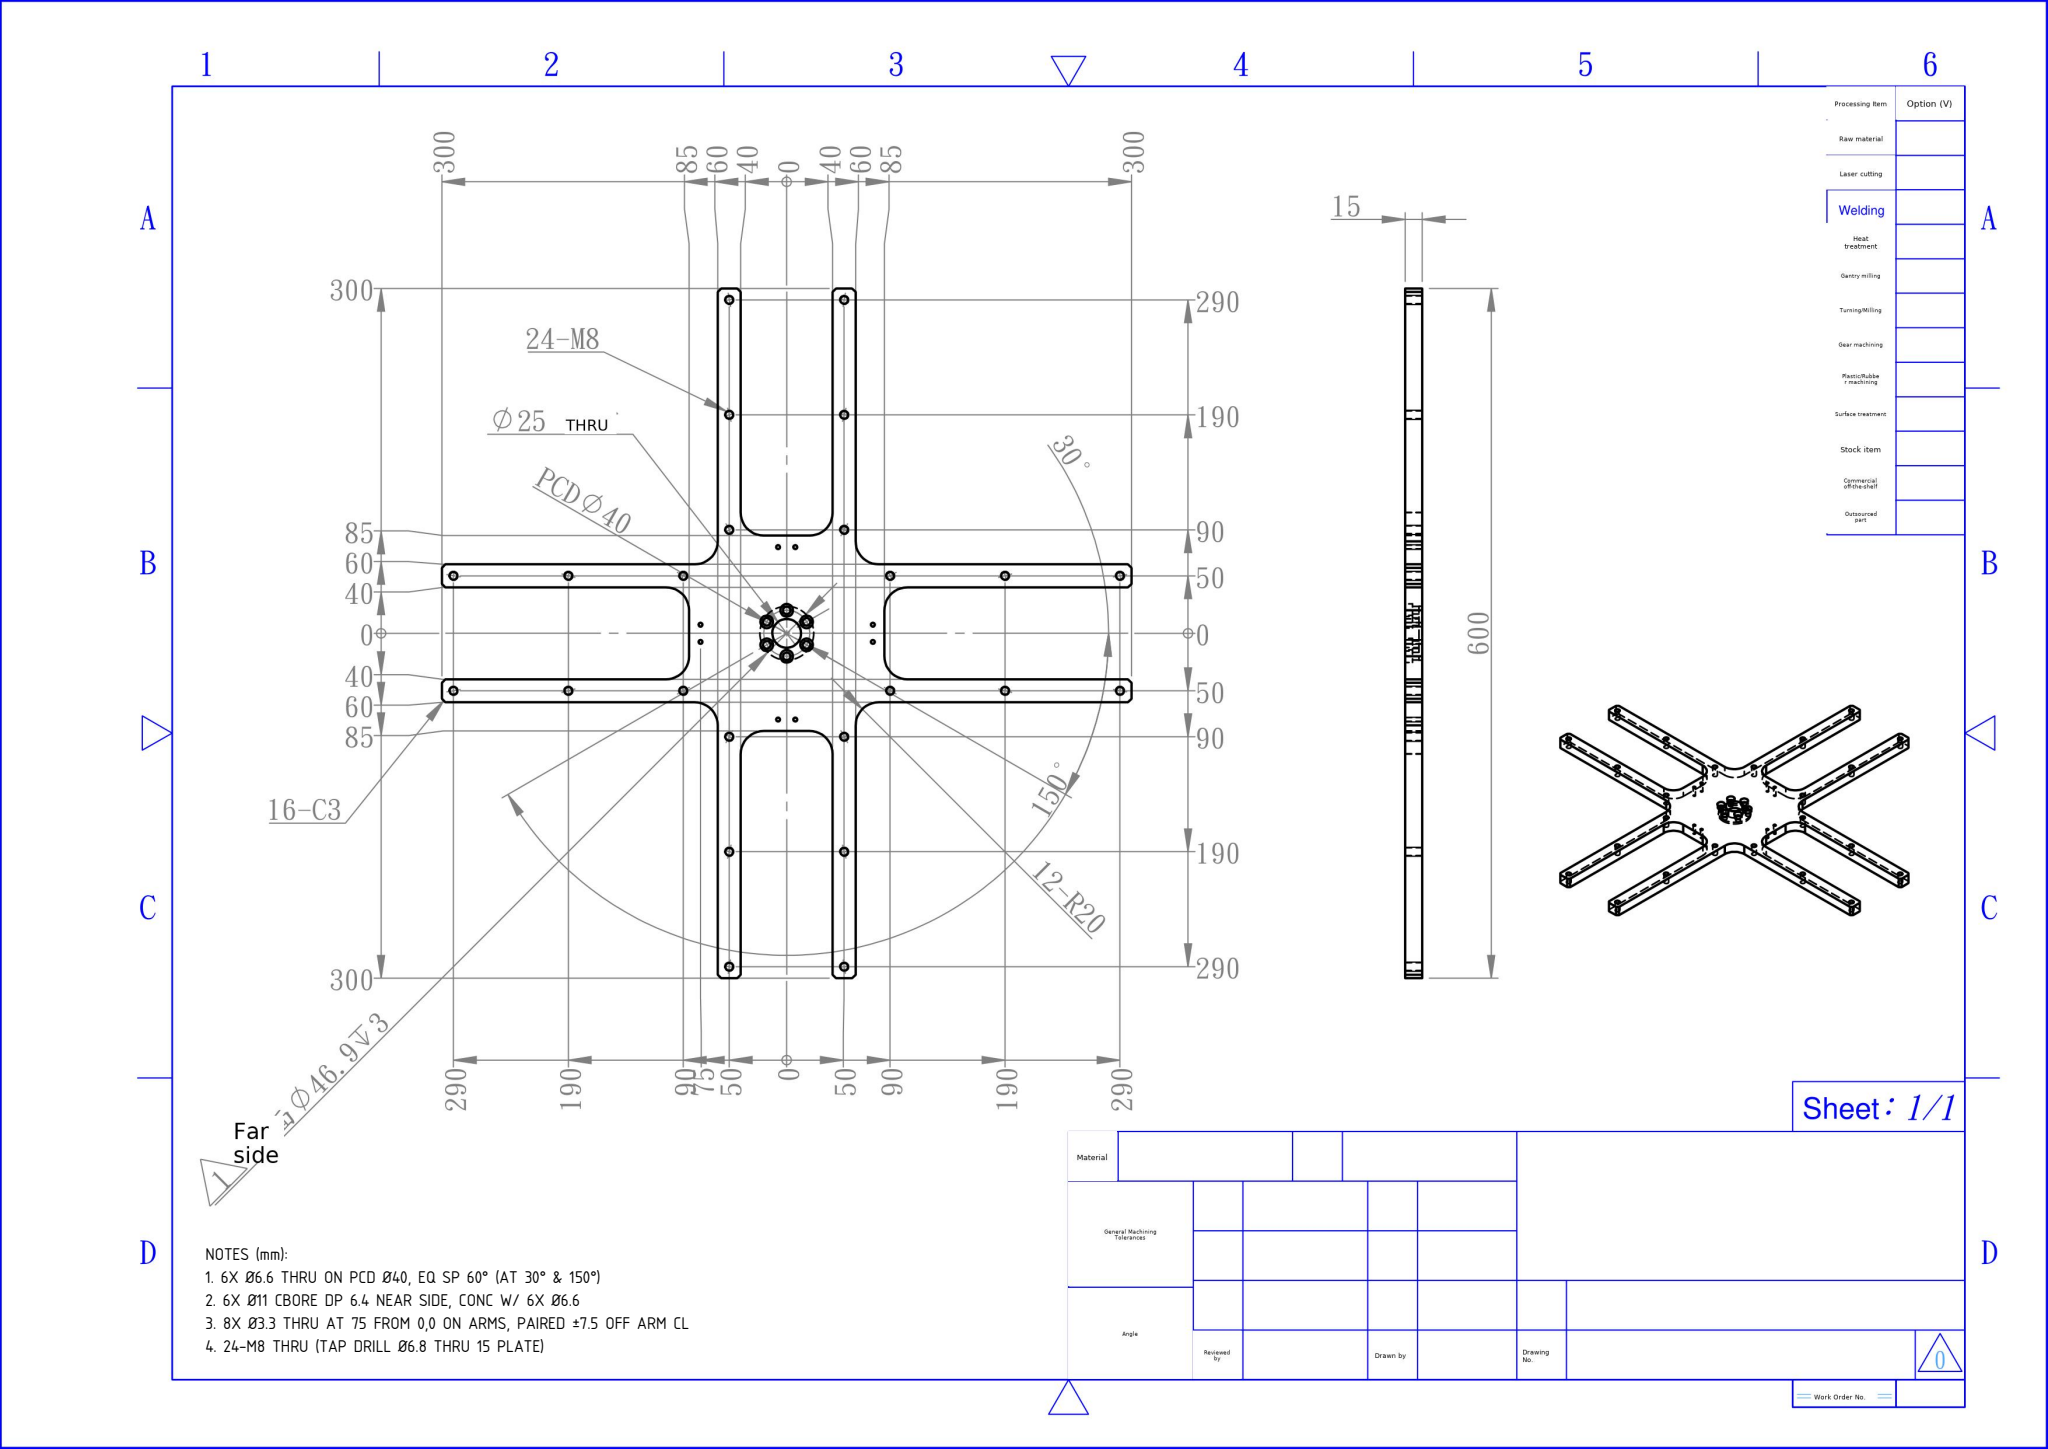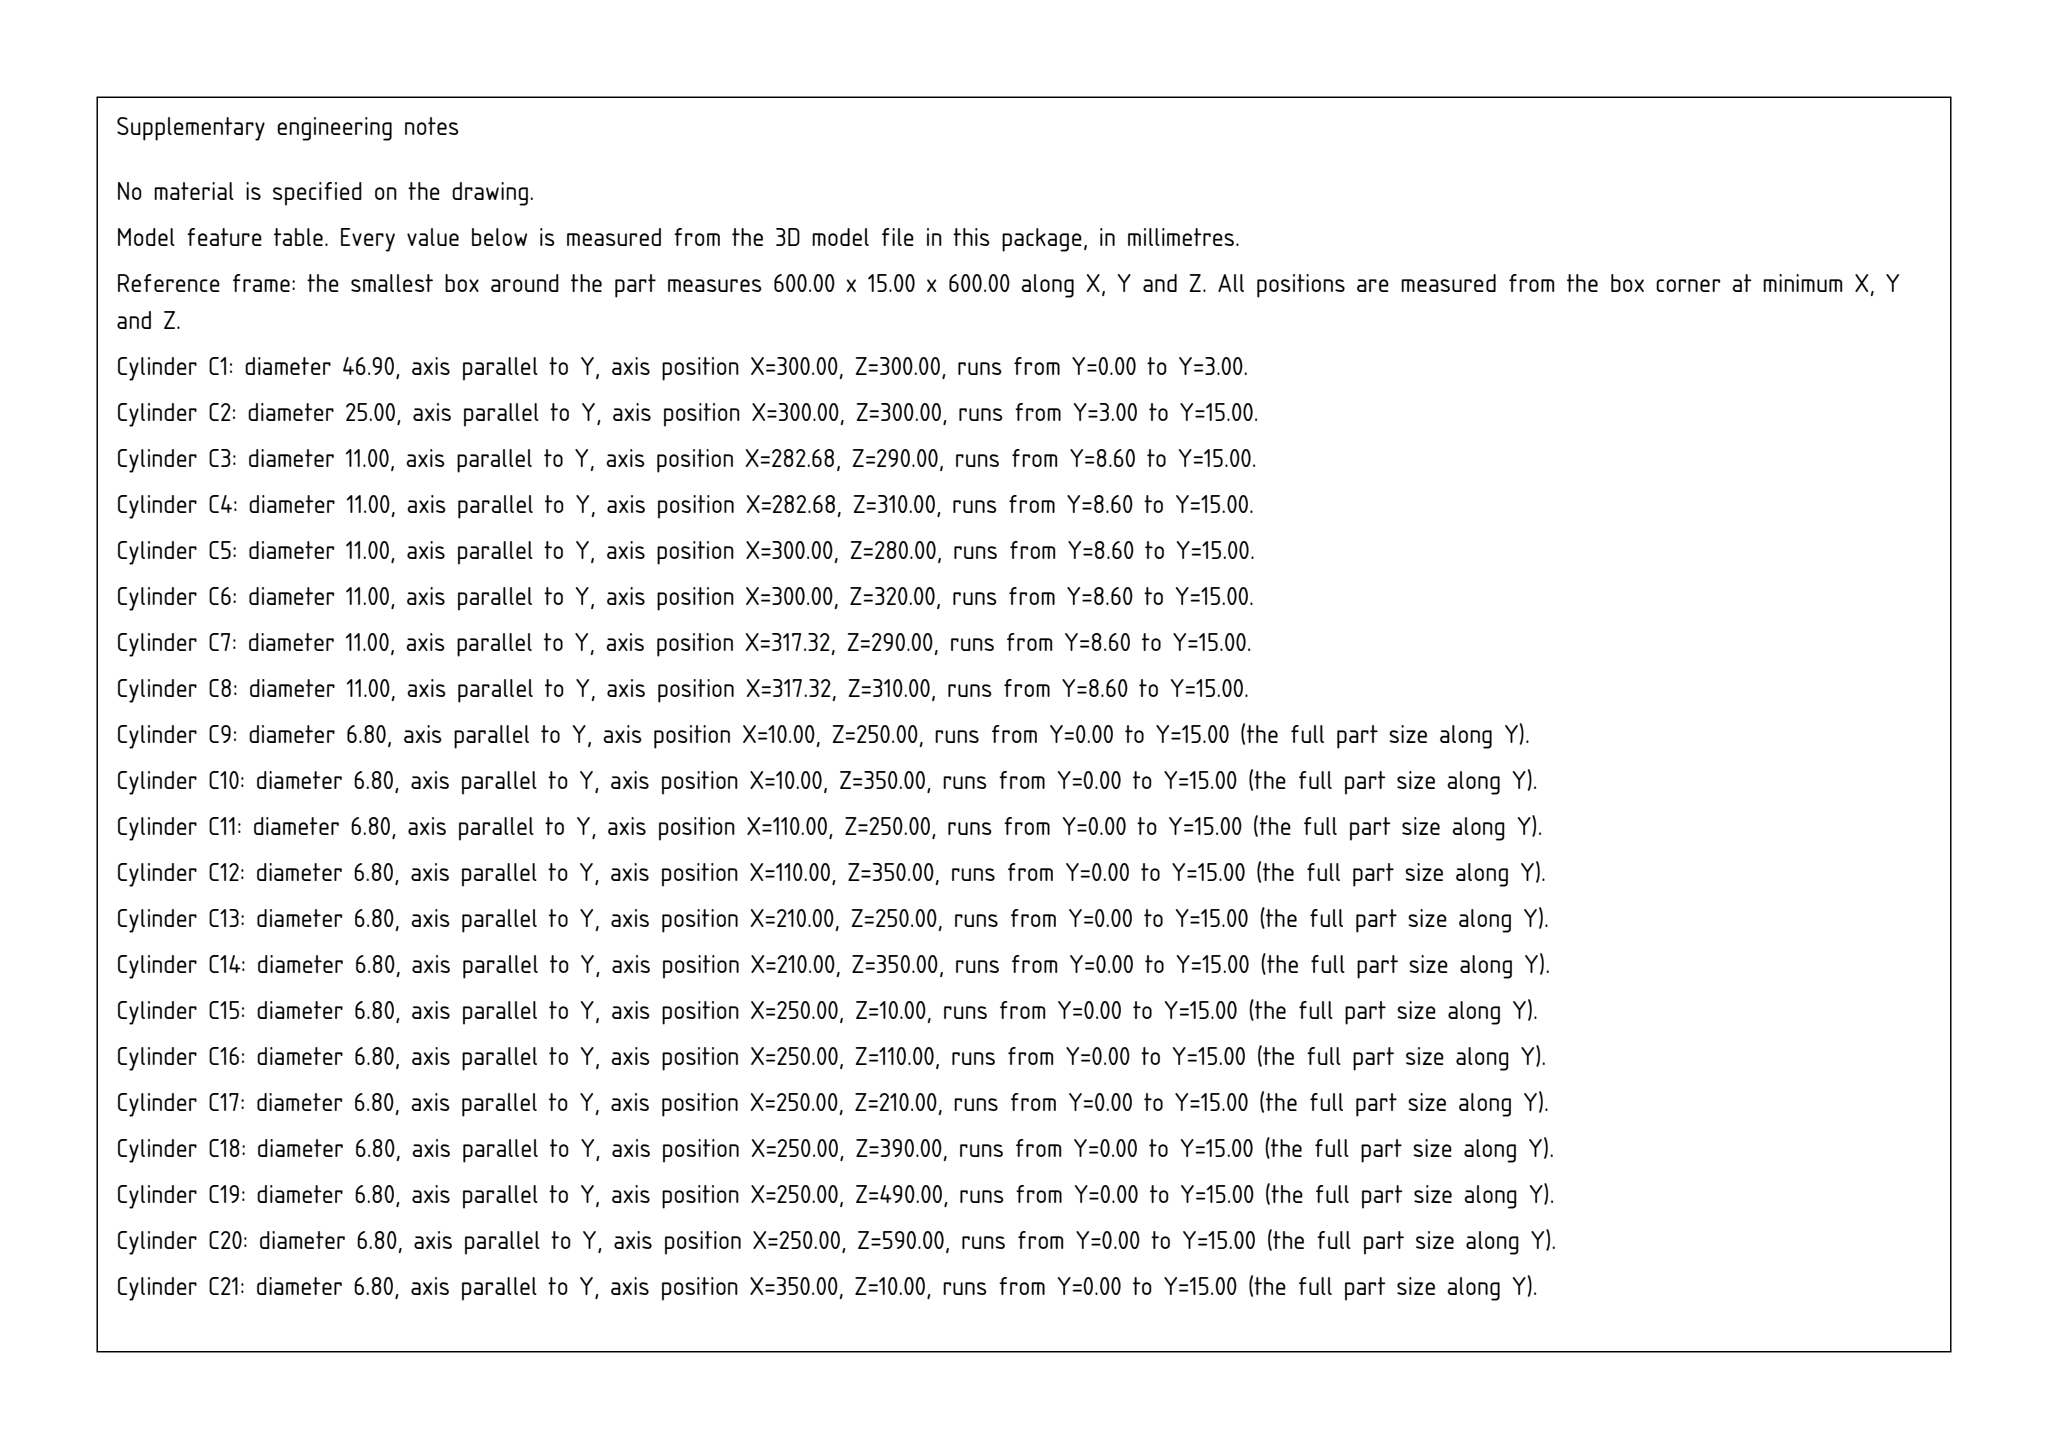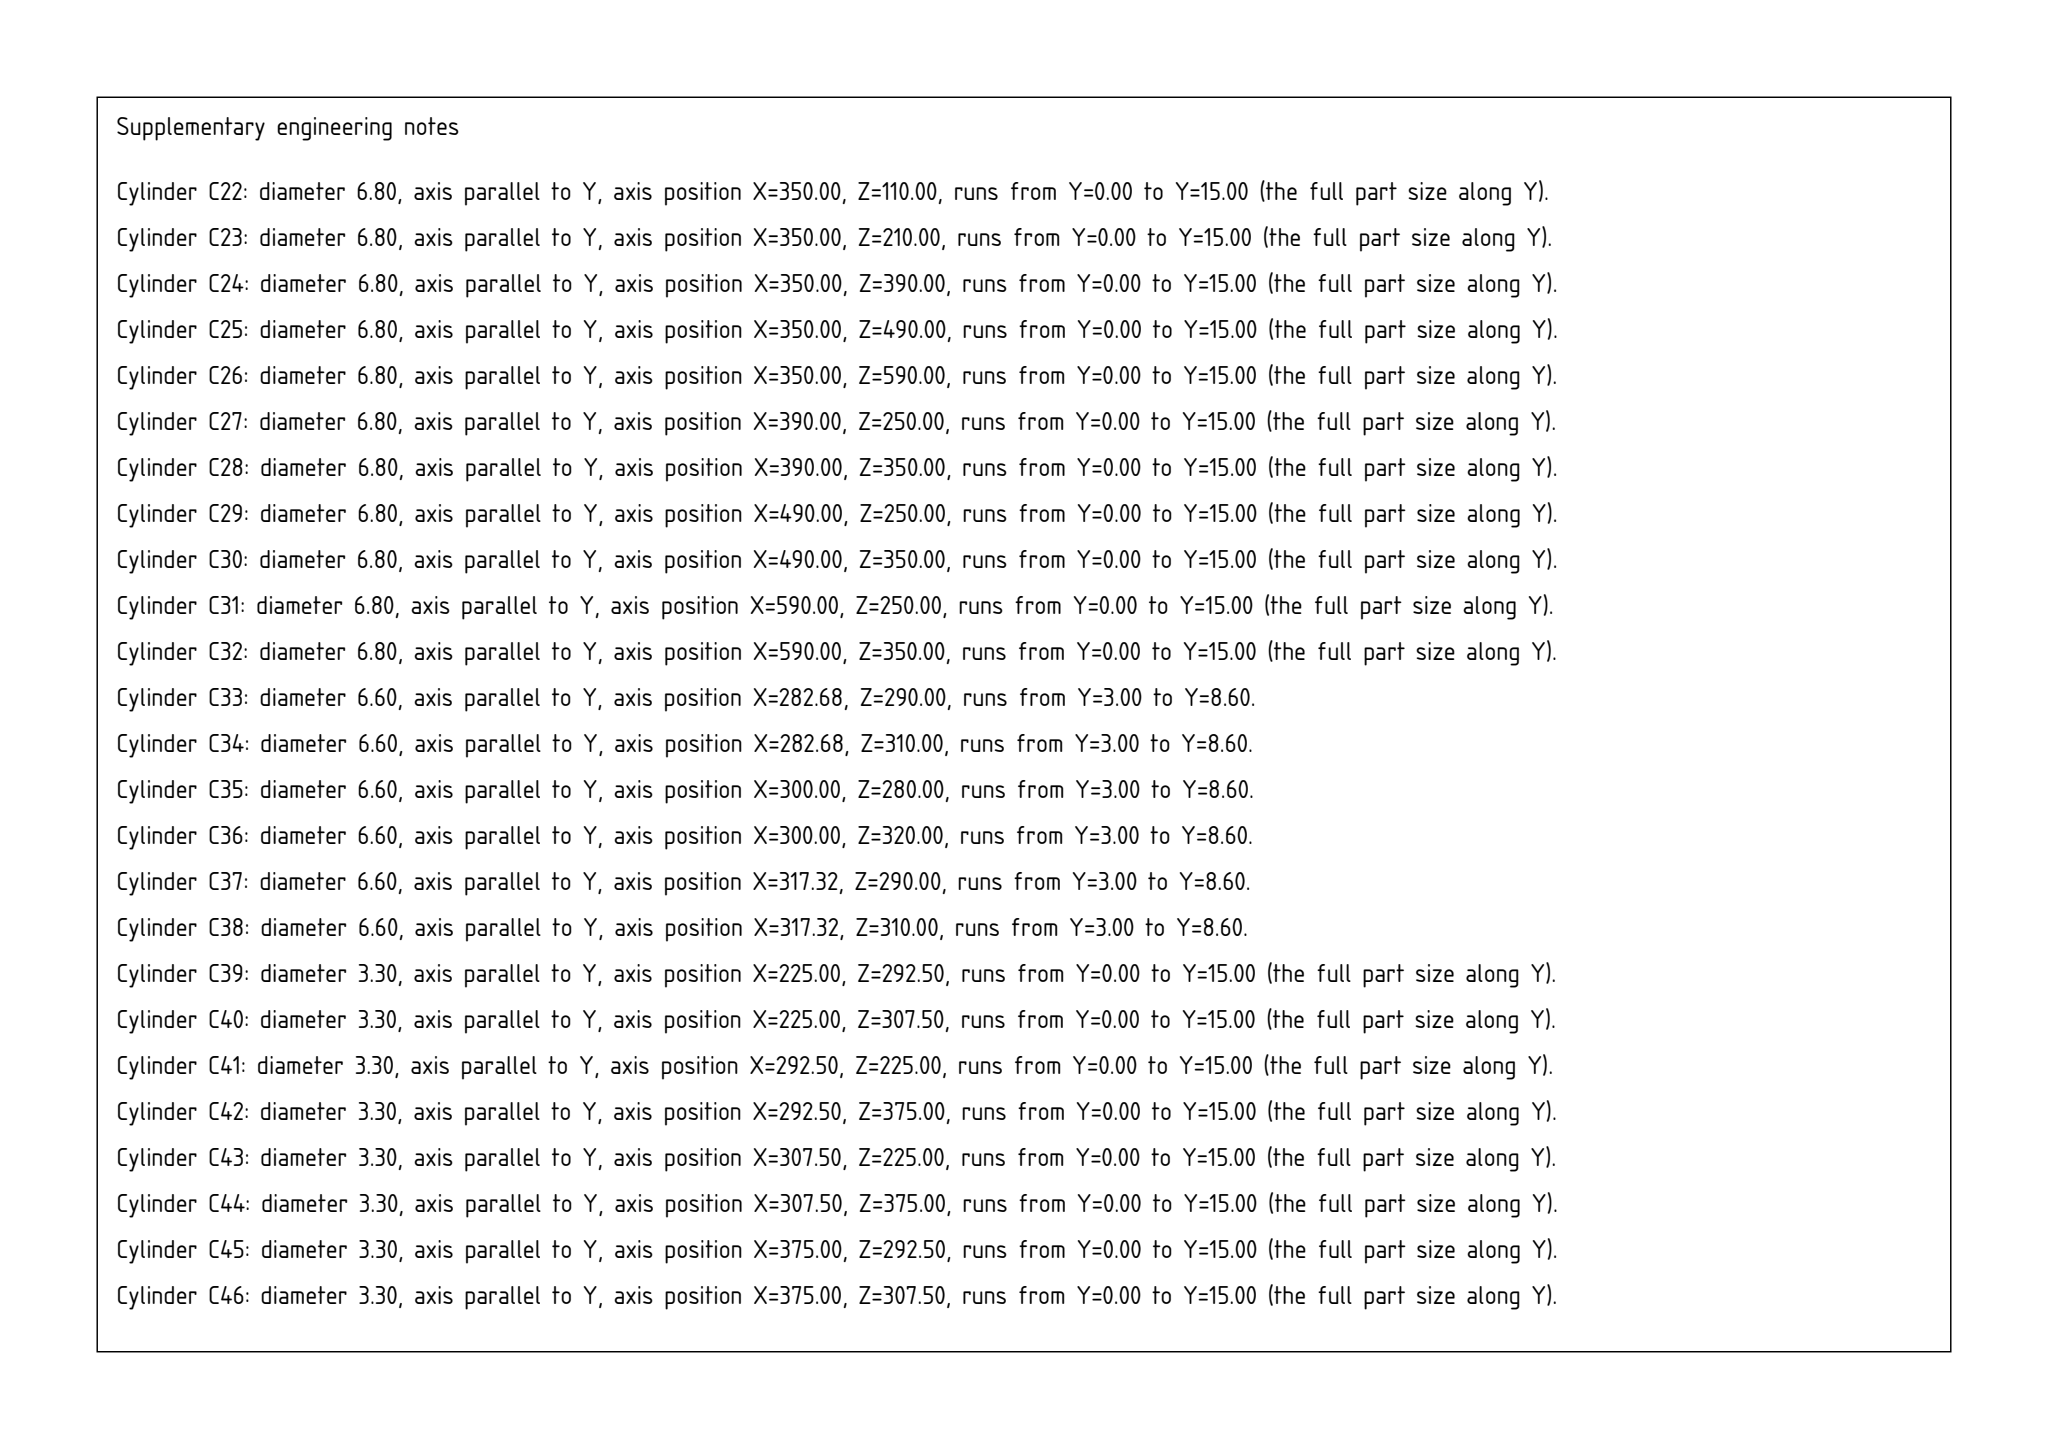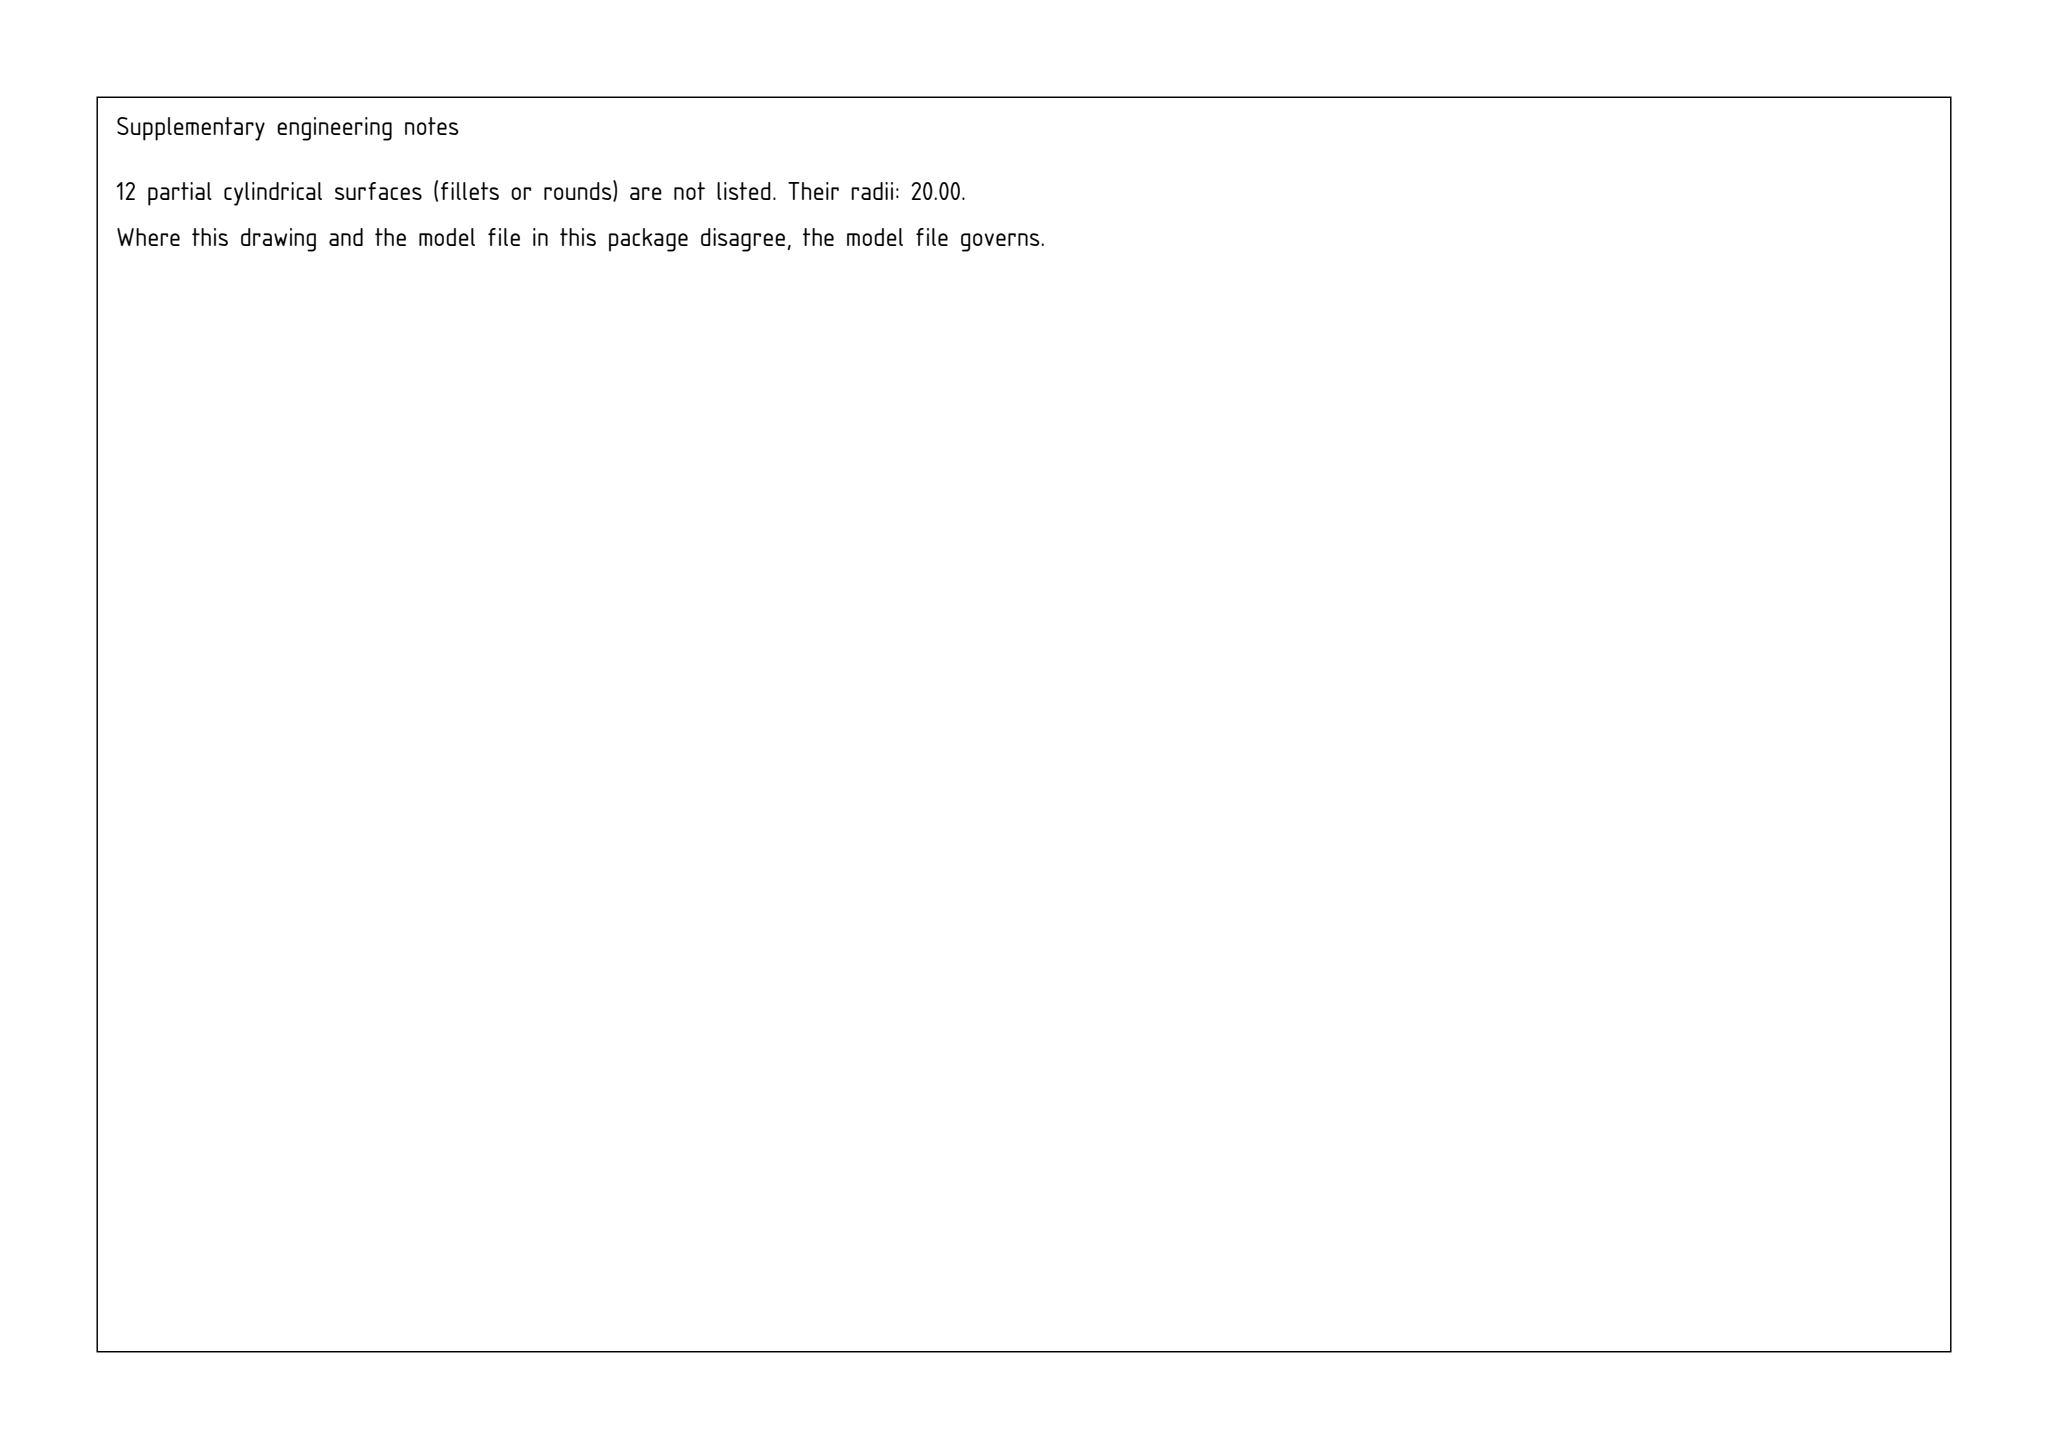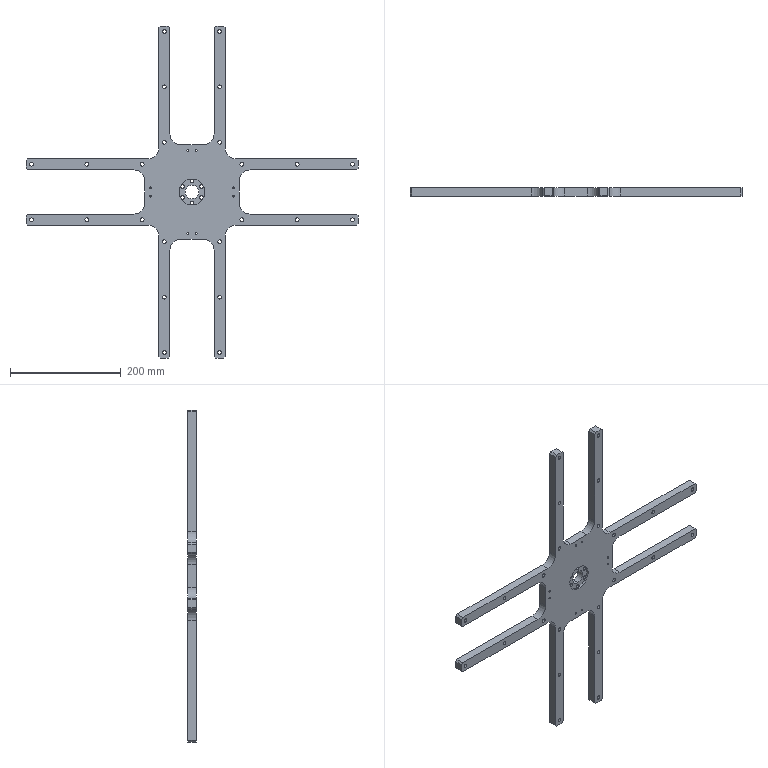Part | SolidWorks | mm | 1 solid | 157 faces | box 600 x 15 x 600 mm | volume 896399 mm3 | cylinder 104 | plane 53 | commonest cylinder face diameters 6.8 x48 3.3 x16 11 x12 6.6 x12 40 x12 25 x2 46.9 x2
Drawing notes:
6X Ø6.6 THRU ON PCD Ø40, EQ SP 60° (AT 30° & 150°) | from the solid: Ø6.6 cyls at (282.68,290),(282.68,310),(300,280),(300,320),(317.32,290),(317.32,310) = R20 about (300,300)
6X Ø11 CBORE DP 6.4 NEAR SIDE, CONC W/ 6X Ø6.6 | from the solid: Ø11 cyls len 6.4 coaxial with the 6X Ø6.6 holes; floor plane y=8.6
8X Ø3.3 THRU AT 75 FROM 0,0 ON ARMS, PAIRED ±7.5 OFF ARM CL | from the solid: Ø3.3 thru cyls (len 15) at x/z 225 & 375 (75 from CL 300) paired at 292.5 & 307.5
24-M8 THRU (TAP DRILL Ø6.8 THRU 15 PLATE) | from the solid: 38 off Ø6.8 cyls, axis y, length 15.0 = full plate thickness (bbox y=15)
build123d program:
from build123d import *

# Parameters (mm, degrees)
BOSS_EXTRUDE1_DEPTH                                  = 15
SKETCH5_R                                            = 23.45
CUT_EXTRUDE2_DEPTH                                   = 3
SKETCH9_R                                            = 12.5
CUT_EXTRUDE6_DEPTH                                   = 425.529
M6_HEX_SOCKET_HEAD_CAP_SCREW_COUNTERBORE_D           = 6.6
M6_HEX_SOCKET_HEAD_CAP_SCREW_COUNTERBORE_CBORE_D     = 11
M6_HEX_SOCKET_HEAD_CAP_SCREW_COUNTERBORE_CBORE_DEPTH = 6.4
CIRCULAR_PATTERN1_COUNT                              = 6
FILLET1_R                                            = 20
CHAMFER1_SIZE                                        = 3
M8_TAPPED_HOLE1_D                                    = 6.8
M4_TAPPED_HOLE1_D                                    = 3.3
CIRCULAR_PATTERN2_COUNT                              = 4


with BuildPart() as part:
    # Sketch1 → Boss-Extrude1 (new body)
    with BuildSketch(Plane(origin=(0, 0, 0), x_dir=(1, 0, 0), z_dir=(0, 1, 0))):
        Polygon((-60, 60), (-60, 300), (-40, 300), (-40, 85), (40, 85), (40, 300), (60, 300), (60, 60), (300, 60), (300, 40), (85, 40), (85, -40), (300, -40), (300, -60), (60, -60), (60, -300), (40, -300), (40, -85), (-40, -85), (-40, -300), (-60, -300), (-60, -60), (-300, -60), (-300, -40), (-85, -40), (-85, 40), (-300, 40), (-300, 60), align=None)
    extrude(amount=BOSS_EXTRUDE1_DEPTH)

    # Sketch5 → Cut-Extrude2 (cut)
    with BuildSketch(Plane(origin=(0, 0, 0), x_dir=(1, 0, 0), z_dir=(0, 1, 0))):
        with Locations(Location((0, 0, 0), (0, 0, 270))):
            Circle(SKETCH5_R)
    extrude(amount=CUT_EXTRUDE2_DEPTH, mode=Mode.SUBTRACT)

    # Sketch9 → Cut-Extrude6 (cut, through all)
    with BuildSketch(Plane.XZ.offset(-15)):
        with Locations(Location((0, 0, 0), (0, 0, 90))):
            Circle(SKETCH9_R)
    extrude(amount=CUT_EXTRUDE6_DEPTH, mode=Mode.SUBTRACT)

    # M6 Hex Socket Head Cap Screw Counterbore (through all)
    with Locations(Plane(origin=(0, 15, 0), x_dir=(1, 0, 0), z_dir=(0, 1, 0))):
        with Locations((0, 20)):
            m6_hex_socket_head_cap_screw_counterbore = CounterBoreHole(M6_HEX_SOCKET_HEAD_CAP_SCREW_COUNTERBORE_D / 2, M6_HEX_SOCKET_HEAD_CAP_SCREW_COUNTERBORE_CBORE_D / 2, M6_HEX_SOCKET_HEAD_CAP_SCREW_COUNTERBORE_CBORE_DEPTH)

    # Circular Pattern1: M6 Hex Socket Head Cap Screw Counterbore ×6 about axis
    circular_pattern1_axis = Axis((0, 0, 0), (0, 1, 0))
    for i in range(1, CIRCULAR_PATTERN1_COUNT):
        add(m6_hex_socket_head_cap_screw_counterbore.rotate(circular_pattern1_axis, i * 360 / CIRCULAR_PATTERN1_COUNT), mode=Mode.SUBTRACT)

    # Fillet1
    fillet1_edges = [part.edges().sort_by_distance(p)[0] for p in [
        (-60, 7.5, -60),
        (-40, 7.5, -85),
        (40, 7.5, -85),
        (60, 7.5, -60),
        (85, 7.5, -40),
        (85, 7.5, 40),
        (60, 7.5, 60),
        (40, 7.5, 85),
        (-40, 7.5, 85),
        (-60, 7.5, 60),
        (-85, 7.5, 40),
        (-85, 7.5, -40),
    ]]
    fillet(fillet1_edges, radius=FILLET1_R)

    # Chamfer1
    chamfer1_edges = [part.edges().sort_by_distance(p)[0] for p in [
        (-60, 7.5, -300),
        (-40, 7.5, -300),
        (40, 7.5, -300),
        (60, 7.5, -300),
        (300, 7.5, -60),
        (300, 7.5, -40),
        (300, 7.5, 40),
        (300, 7.5, 60),
        (60, 7.5, 300),
        (40, 7.5, 300),
        (-40, 7.5, 300),
        (-60, 7.5, 300),
        (-300, 7.5, 60),
        (-300, 7.5, 40),
        (-300, 7.5, -40),
        (-300, 7.5, -60),
    ]]
    chamfer(chamfer1_edges, length=CHAMFER1_SIZE)

    # M8 Tapped Hole1 (through all)
    with Locations(Plane(origin=(0, 15, 0), x_dir=(1, 0, 0), z_dir=(0, 1, 0))):
        with Locations((-290, 50), (-190, 50), (-90, 50), (-90, -50), (-190, -50), (-290, -50)):
            m8_tapped_hole1 = Hole(M8_TAPPED_HOLE1_D / 2)

    # M4 Tapped Hole1 (through all)
    with Locations(Plane(origin=(0, 15, 0), x_dir=(1, 0, 0), z_dir=(0, 1, 0))):
        with Locations((-75, -7.5), (-75, 7.5)):
            m4_tapped_hole1 = Hole(M4_TAPPED_HOLE1_D / 2)

    # Circular Pattern2: M8 Tapped Hole1, M4 Tapped Hole1 ×4 about axis
    circular_pattern2_axis = Axis((0, 0, 0), (0, 1, 0))
    add([m8_tapped_hole1.rotate(circular_pattern2_axis, i * 360 / CIRCULAR_PATTERN2_COUNT) for i in range(1, CIRCULAR_PATTERN2_COUNT)], mode=Mode.SUBTRACT)
    add([m4_tapped_hole1.rotate(circular_pattern2_axis, i * 360 / CIRCULAR_PATTERN2_COUNT) for i in range(1, CIRCULAR_PATTERN2_COUNT)], mode=Mode.SUBTRACT)


solid = part.part